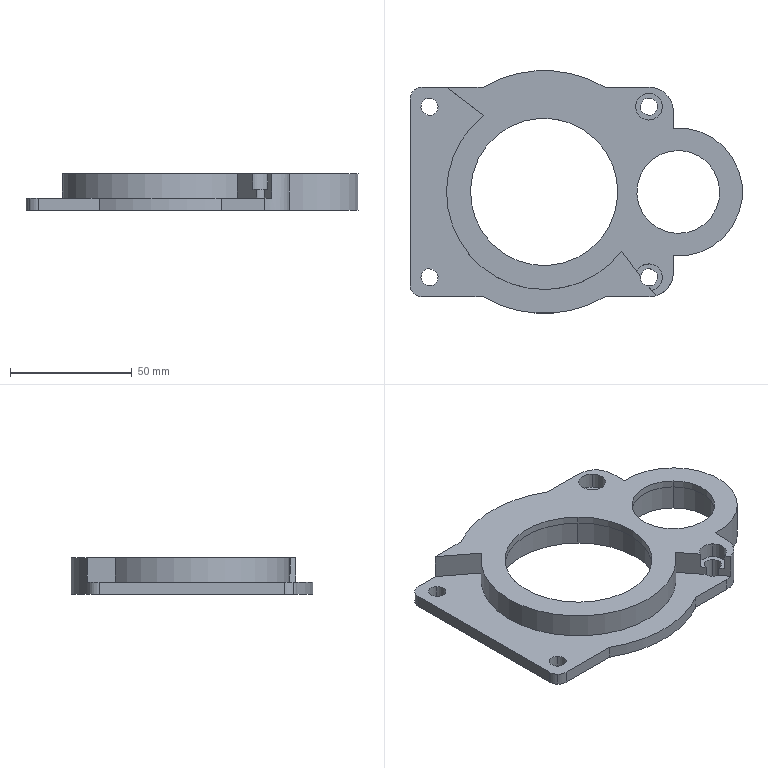Component | SolidWorks | DriveDevice-1_ProtectivePlate-1 | 1 solid | 46 faces | volume 69324 mm3 | cylinder 29 | plane 17 | commonest cylinder face diameters 7 x8 11 x4 10 x3 60.4 x2 34 x2 38 x2 66 x2 99.5 x2